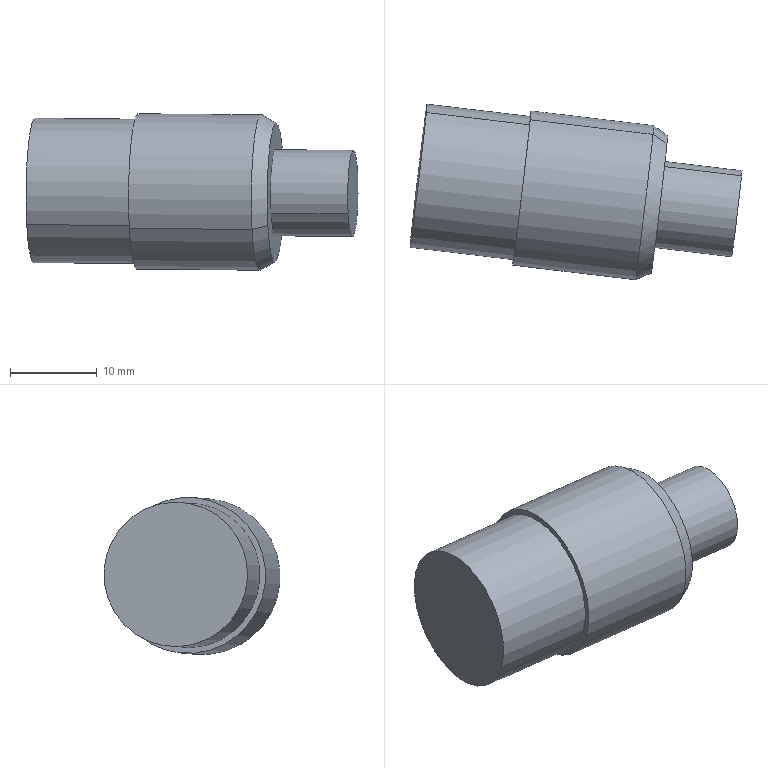Component | SolidWorks | White-1 | 1 solid | 12 faces | box 38.32 x 20.33 x 18.14 mm | volume 7353 mm3 | cylinder 6 | plane 4 | cone 2 | commonest cylinder face diameters 16.68 x2 10 x2 18 x2
build123d program:
from build123d import *

# Parameters (mm, degrees)
SKETCH1_R           = 5
BOSS_EXTRUDE1_DEPTH = 9
SKETCH2_R           = 9
BOSS_EXTRUDE2_DEPTH = 18
CHAMFER1_SIZE       = 1
CHAMFER1_SIZE2      = 1.732
CUT_EXTRUDE1_START  = -2
SKETCH3_R           = 9
SKETCH3_R_2         = 8.34
CUT_EXTRUDE1_DEPTH  = 2
SKETCH4_R           = 8.34
BOSS_EXTRUDE3_DEPTH = 10


with BuildPart() as part:
    # Sketch1 → Boss-Extrude1 (new body)
    with BuildSketch(Plane.XY):
        Circle(SKETCH1_R)
    extrude(amount=BOSS_EXTRUDE1_DEPTH)

    # Sketch2 → Boss-Extrude2 (add)
    with BuildSketch(Plane.XY.offset(9)):
        Circle(SKETCH2_R)
    extrude(amount=BOSS_EXTRUDE2_DEPTH)

    # Chamfer1
    chamfer1_edges = [part.edges().sort_by_distance(p)[0] for p in [
        (-9, 0, 9),
    ]]
    chamfer1_side = [part.faces().sort_by_distance(p)[0] for p in [
        (-8.745, 0, 9),
    ]]
    chamfer(chamfer1_edges, length=CHAMFER1_SIZE, length2=CHAMFER1_SIZE2, reference=chamfer1_side[0])

    # Sketch3 → Cut-Extrude1 (cut)
    with BuildSketch(Plane.XY.offset(27).offset(CUT_EXTRUDE1_START)):
        Circle(SKETCH3_R)
        Circle(SKETCH3_R_2, mode=Mode.SUBTRACT)
    extrude(amount=CUT_EXTRUDE1_DEPTH, mode=Mode.SUBTRACT)

    # Sketch4 → Boss-Extrude3 (add)
    with BuildSketch(Plane.XY.offset(27)):
        Circle(SKETCH4_R)
    extrude(amount=BOSS_EXTRUDE3_DEPTH)


solid = part.part

# Placed as in the assembly
solid = solid.moved(Location((-29.102, 70.681, -1.561), (-85.302, -83.182, 96.374)))
STEP:
#1=COLOUR_RGB('',0.7922,0.8196,0.9333);
#2=FILL_AREA_STYLE_COLOUR('',#1);
#3=FILL_AREA_STYLE('',(#2));
#4=SURFACE_STYLE_FILL_AREA(#3);
#5=SURFACE_SIDE_STYLE('',(#4));
#6=SURFACE_STYLE_USAGE(.BOTH.,#5);
#7=PRESENTATION_STYLE_ASSIGNMENT((#6));
#8=CARTESIAN_POINT('',(-2.087,3.186,0.1035));
#9=VERTEX_POINT('',#8);
#10=CARTESIAN_POINT('',(-2.159,2.612,-0.2072));
#11=VERTEX_POINT('',#10);
#12=CARTESIAN_POINT('',(-2.123,2.899,-0.05188));
#13=DIRECTION('',(-0.9929,0.1183,0.009724));
#14=DIRECTION('',(0.1088,0.8743,0.4731));
#15=AXIS2_PLACEMENT_3D('',#12,#13,#14);
#16=CIRCLE('',#15,0.3283);
#17=EDGE_CURVE('',#9,#11,#16,.T.);
#18=ORIENTED_EDGE('',*,*,#17,.T.);
#19=CARTESIAN_POINT('',(-2.628,2.668,-0.2026));
#20=VERTEX_POINT('',#19);
#21=CARTESIAN_POINT('',(-2.159,2.612,-0.2072));
#22=DIRECTION('',(-0.9929,0.1183,0.009724));
#23=VECTOR('',#22,39.37);
#24=LINE('',#21,#23);
#25=EDGE_CURVE('',#11,#20,#24,.T.);
#26=ORIENTED_EDGE('',*,*,#25,.T.);
#27=CARTESIAN_POINT('',(-2.556,3.242,0.108));
#28=VERTEX_POINT('',#27);
#29=CARTESIAN_POINT('',(-2.592,2.955,-0.04729));
#30=DIRECTION('',(-0.9929,0.1183,0.009724));
#31=DIRECTION('',(0.1088,0.8743,0.4731));
#32=AXIS2_PLACEMENT_3D('',#29,#30,#31);
#33=CIRCLE('',#32,0.3283);
#34=EDGE_CURVE('',#28,#20,#33,.T.);
#35=ORIENTED_EDGE('',*,*,#34,.F.);
#36=CARTESIAN_POINT('',(-2.087,3.186,0.1035));
#37=DIRECTION('',(-0.9929,0.1183,0.009724));
#38=VECTOR('',#37,39.37);
#39=LINE('',#36,#38);
#40=EDGE_CURVE('',#9,#28,#39,.T.);
#41=ORIENTED_EDGE('',*,*,#40,.F.);
#42=EDGE_LOOP('',(#18,#26,#35,#41));
#43=FACE_OUTER_BOUND('',#42,.T.);
#44=CARTESIAN_POINT('',(-2.123,2.899,-0.05188));
#45=DIRECTION('',(-0.9929,0.1183,0.009724));
#46=DIRECTION('',(0.1088,0.8743,0.4731));
#47=AXIS2_PLACEMENT_3D('',#44,#45,#46);
#48=CYLINDRICAL_SURFACE('',#47,0.3283);
#49=ADVANCED_FACE('',(#43),#48,.T.);
#50=CARTESIAN_POINT('',(-1.532,2.549,-0.207));
#51=VERTEX_POINT('',#50);
#52=CARTESIAN_POINT('',(-1.463,3.1,0.091));
#53=VERTEX_POINT('',#52);
#54=CARTESIAN_POINT('',(-1.498,2.825,-0.05801));
#55=DIRECTION('',(0.9929,-0.1183,-0.009724));
#56=DIRECTION('',(0.1088,0.8743,0.4731));
#57=AXIS2_PLACEMENT_3D('',#54,#55,#56);
#58=CIRCLE('',#57,0.315);
#59=EDGE_CURVE('',#51,#53,#58,.T.);
#60=ORIENTED_EDGE('',*,*,#59,.F.);
#61=CARTESIAN_POINT('',(-1.604,2.523,-0.225));
#62=VERTEX_POINT('',#61);
#63=CARTESIAN_POINT('',(-1.604,2.523,-0.225));
#64=DIRECTION('',(-0.9143,-0.3347,-0.2281));
#65=VECTOR('',#64,39.37);
#66=LINE('',#63,#65);
#67=EDGE_CURVE('',#51,#62,#66,.T.);
#68=ORIENTED_EDGE('',*,*,#67,.T.);
#69=CARTESIAN_POINT('',(-1.527,3.143,0.1103));
#70=VERTEX_POINT('',#69);
#71=CARTESIAN_POINT('',(-1.565,2.833,-0.05735));
#72=DIRECTION('',(-0.9929,0.1183,0.009724));
#73=DIRECTION('',(0.1088,0.8743,0.4731));
#74=AXIS2_PLACEMENT_3D('',#71,#72,#73);
#75=CIRCLE('',#74,0.3543);
#76=EDGE_CURVE('',#70,#62,#75,.T.);
#77=ORIENTED_EDGE('',*,*,#76,.F.);
#78=CARTESIAN_POINT('',(-1.527,3.143,0.1103));
#79=DIRECTION('',(-0.8055,0.5396,0.245));
#80=VECTOR('',#79,39.37);
#81=LINE('',#78,#80);
#82=EDGE_CURVE('',#53,#70,#81,.T.);
#83=ORIENTED_EDGE('',*,*,#82,.F.);
#84=EDGE_LOOP('',(#60,#68,#77,#83));
#85=FACE_OUTER_BOUND('',#84,.T.);
#86=CARTESIAN_POINT('',(-1.565,2.833,-0.05735));
#87=DIRECTION('',(-0.9929,0.1183,0.009724));
#88=DIRECTION('',(0.1088,0.8743,0.4731));
#89=AXIS2_PLACEMENT_3D('',#86,#87,#88);
#90=CONICAL_SURFACE('',#89,0.3543,0.5236);
#91=ADVANCED_FACE('',(#85),#90,.T.);
#92=CARTESIAN_POINT('',(-1.476,2.997,0.03512));
#93=VERTEX_POINT('',#92);
#94=CARTESIAN_POINT('',(-1.519,2.653,-0.1511));
#95=VERTEX_POINT('',#94);
#96=CARTESIAN_POINT('',(-1.498,2.825,-0.05801));
#97=DIRECTION('',(-0.9929,0.1183,0.009724));
#98=DIRECTION('',(0.1088,0.8743,0.4731));
#99=AXIS2_PLACEMENT_3D('',#96,#97,#98);
#100=CIRCLE('',#99,0.1969);
#101=EDGE_CURVE('',#93,#95,#100,.T.);
#102=ORIENTED_EDGE('',*,*,#101,.F.);
#103=CARTESIAN_POINT('',(-1.124,2.955,0.03167));
#104=VERTEX_POINT('',#103);
#105=CARTESIAN_POINT('',(-1.476,2.997,0.03512));
#106=DIRECTION('',(0.9929,-0.1183,-0.009724));
#107=VECTOR('',#106,39.37);
#108=LINE('',#105,#107);
#109=EDGE_CURVE('',#93,#104,#108,.T.);
#110=ORIENTED_EDGE('',*,*,#109,.T.);
#111=CARTESIAN_POINT('',(-1.167,2.611,-0.1546));
#112=VERTEX_POINT('',#111);
#113=CARTESIAN_POINT('',(-1.146,2.783,-0.06145));
#114=DIRECTION('',(-0.9929,0.1183,0.009724));
#115=DIRECTION('',(0.1088,0.8743,0.4731));
#116=AXIS2_PLACEMENT_3D('',#113,#114,#115);
#117=CIRCLE('',#116,0.1969);
#118=EDGE_CURVE('',#104,#112,#117,.T.);
#119=ORIENTED_EDGE('',*,*,#118,.T.);
#120=CARTESIAN_POINT('',(-1.519,2.653,-0.1511));
#121=DIRECTION('',(0.9929,-0.1183,-0.009724));
#122=VECTOR('',#121,39.37);
#123=LINE('',#120,#122);
#124=EDGE_CURVE('',#95,#112,#123,.T.);
#125=ORIENTED_EDGE('',*,*,#124,.F.);
#126=EDGE_LOOP('',(#102,#110,#119,#125));
#127=FACE_OUTER_BOUND('',#126,.T.);
#128=CARTESIAN_POINT('',(-1.498,2.825,-0.05801));
#129=DIRECTION('',(0.9929,-0.1183,-0.009724));
#130=DIRECTION('',(-0.1088,-0.8743,-0.4731));
#131=AXIS2_PLACEMENT_3D('',#128,#129,#130);
#132=CYLINDRICAL_SURFACE('',#131,0.1969);
#133=ADVANCED_FACE('',(#127),#132,.T.);
#134=CARTESIAN_POINT('',(-2.084,3.209,0.1157));
#135=VERTEX_POINT('',#134);
#136=CARTESIAN_POINT('',(-2.162,2.589,-0.2195));
#137=VERTEX_POINT('',#136);
#138=CARTESIAN_POINT('',(-2.123,2.899,-0.05188));
#139=DIRECTION('',(-0.9929,0.1183,0.009724));
#140=DIRECTION('',(0.1088,0.8743,0.4731));
#141=AXIS2_PLACEMENT_3D('',#138,#139,#140);
#142=CIRCLE('',#141,0.3543);
#143=EDGE_CURVE('',#135,#137,#142,.T.);
#144=ORIENTED_EDGE('',*,*,#143,.F.);
#145=CARTESIAN_POINT('',(-2.163,3.218,0.1165));
#146=DIRECTION('',(0.9929,-0.1183,-0.009724));
#147=VECTOR('',#146,39.37);
#148=LINE('',#145,#147);
#149=EDGE_CURVE('',#135,#70,#148,.T.);
#150=ORIENTED_EDGE('',*,*,#149,.T.);
#151=ORIENTED_EDGE('',*,*,#76,.T.);
#152=CARTESIAN_POINT('',(-2.24,2.599,-0.2187));
#153=DIRECTION('',(0.9929,-0.1183,-0.009724));
#154=VECTOR('',#153,39.37);
#155=LINE('',#152,#154);
#156=EDGE_CURVE('',#137,#62,#155,.T.);
#157=ORIENTED_EDGE('',*,*,#156,.F.);
#158=EDGE_LOOP('',(#144,#150,#151,#157));
#159=FACE_OUTER_BOUND('',#158,.T.);
#160=CARTESIAN_POINT('',(-2.201,2.909,-0.05112));
#161=DIRECTION('',(0.9929,-0.1183,-0.009724));
#162=DIRECTION('',(-0.1088,-0.8743,-0.4731));
#163=AXIS2_PLACEMENT_3D('',#160,#161,#162);
#164=CYLINDRICAL_SURFACE('',#163,0.3543);
#165=ADVANCED_FACE('',(#159),#164,.T.);
#166=ORIENTED_EDGE('',*,*,#149,.F.);
#167=CARTESIAN_POINT('',(-2.123,2.899,-0.05188));
#168=DIRECTION('',(-0.9929,0.1183,0.009724));
#169=DIRECTION('',(0.1088,0.8743,0.4731));
#170=AXIS2_PLACEMENT_3D('',#167,#168,#169);
#171=CIRCLE('',#170,0.3543);
#172=EDGE_CURVE('',#137,#135,#171,.T.);
#173=ORIENTED_EDGE('',*,*,#172,.F.);
#174=ORIENTED_EDGE('',*,*,#156,.T.);
#175=CARTESIAN_POINT('',(-1.565,2.833,-0.05735));
#176=DIRECTION('',(-0.9929,0.1183,0.009724));
#177=DIRECTION('',(0.1088,0.8743,0.4731));
#178=AXIS2_PLACEMENT_3D('',#175,#176,#177);
#179=CIRCLE('',#178,0.3543);
#180=EDGE_CURVE('',#62,#70,#179,.T.);
#181=ORIENTED_EDGE('',*,*,#180,.T.);
#182=EDGE_LOOP('',(#166,#173,#174,#181));
#183=FACE_OUTER_BOUND('',#182,.T.);
#184=CARTESIAN_POINT('',(-2.201,2.909,-0.05112));
#185=DIRECTION('',(0.9929,-0.1183,-0.009724));
#186=DIRECTION('',(-0.1088,-0.8743,-0.4731));
#187=AXIS2_PLACEMENT_3D('',#184,#185,#186);
#188=CYLINDRICAL_SURFACE('',#187,0.3543);
#189=ADVANCED_FACE('',(#183),#188,.T.);
#190=ORIENTED_EDGE('',*,*,#109,.F.);
#191=CARTESIAN_POINT('',(-1.498,2.825,-0.05801));
#192=DIRECTION('',(-0.9929,0.1183,0.009724));
#193=DIRECTION('',(0.1088,0.8743,0.4731));
#194=AXIS2_PLACEMENT_3D('',#191,#192,#193);
#195=CIRCLE('',#194,0.1969);
#196=EDGE_CURVE('',#95,#93,#195,.T.);
#197=ORIENTED_EDGE('',*,*,#196,.F.);
#198=ORIENTED_EDGE('',*,*,#124,.T.);
#199=CARTESIAN_POINT('',(-1.146,2.783,-0.06145));
#200=DIRECTION('',(-0.9929,0.1183,0.009724));
#201=DIRECTION('',(0.1088,0.8743,0.4731));
#202=AXIS2_PLACEMENT_3D('',#199,#200,#201);
#203=CIRCLE('',#202,0.1969);
#204=EDGE_CURVE('',#112,#104,#203,.T.);
#205=ORIENTED_EDGE('',*,*,#204,.T.);
#206=EDGE_LOOP('',(#190,#197,#198,#205));
#207=FACE_OUTER_BOUND('',#206,.T.);
#208=CARTESIAN_POINT('',(-1.498,2.825,-0.05801));
#209=DIRECTION('',(0.9929,-0.1183,-0.009724));
#210=DIRECTION('',(-0.1088,-0.8743,-0.4731));
#211=AXIS2_PLACEMENT_3D('',#208,#209,#210);
#212=CYLINDRICAL_SURFACE('',#211,0.1969);
#213=ADVANCED_FACE('',(#207),#212,.T.);
#214=ORIENTED_EDGE('',*,*,#204,.F.);
#215=ORIENTED_EDGE('',*,*,#118,.F.);
#216=EDGE_LOOP('',(#214,#215));
#217=FACE_OUTER_BOUND('',#216,.T.);
#218=CARTESIAN_POINT('',(-1.146,2.783,-0.06145));
#219=DIRECTION('',(-0.9929,0.1183,0.009724));
#220=DIRECTION('',(0.1088,0.8743,0.4731));
#221=AXIS2_PLACEMENT_3D('',#218,#219,#220);
#222=PLANE('',#221);
#223=ADVANCED_FACE('',(#217),#222,.F.);
#224=CARTESIAN_POINT('',(-1.498,2.825,-0.05801));
#225=DIRECTION('',(0.9929,-0.1183,-0.009724));
#226=DIRECTION('',(0.1088,0.8743,0.4731));
#227=AXIS2_PLACEMENT_3D('',#224,#225,#226);
#228=CIRCLE('',#227,0.315);
#229=EDGE_CURVE('',#53,#51,#228,.T.);
#230=ORIENTED_EDGE('',*,*,#229,.T.);
#231=ORIENTED_EDGE('',*,*,#59,.T.);
#232=EDGE_LOOP('',(#230,#231));
#233=FACE_OUTER_BOUND('',#232,.T.);
#234=ORIENTED_EDGE('',*,*,#196,.T.);
#235=ORIENTED_EDGE('',*,*,#101,.T.);
#236=EDGE_LOOP('',(#234,#235));
#237=FACE_BOUND('',#236,.T.);
#238=CARTESIAN_POINT('',(-1.498,2.825,-0.05801));
#239=DIRECTION('',(-0.9929,0.1183,0.009724));
#240=DIRECTION('',(0.1088,0.8743,0.4731));
#241=AXIS2_PLACEMENT_3D('',#238,#239,#240);
#242=PLANE('',#241);
#243=ADVANCED_FACE('',(#233,#237),#242,.F.);
#244=ORIENTED_EDGE('',*,*,#67,.F.);
#245=ORIENTED_EDGE('',*,*,#229,.F.);
#246=ORIENTED_EDGE('',*,*,#82,.T.);
#247=ORIENTED_EDGE('',*,*,#180,.F.);
#248=EDGE_LOOP('',(#244,#245,#246,#247));
#249=FACE_OUTER_BOUND('',#248,.T.);
#250=CARTESIAN_POINT('',(-1.565,2.833,-0.05735));
#251=DIRECTION('',(-0.9929,0.1183,0.009724));
#252=DIRECTION('',(0.1088,0.8743,0.4731));
#253=AXIS2_PLACEMENT_3D('',#250,#251,#252);
#254=CONICAL_SURFACE('',#253,0.3543,0.5236);
#255=ADVANCED_FACE('',(#249),#254,.T.);
#256=ORIENTED_EDGE('',*,*,#17,.F.);
#257=CARTESIAN_POINT('',(-2.123,2.899,-0.05188));
#258=DIRECTION('',(-0.9929,0.1183,0.009724));
#259=DIRECTION('',(0.1088,0.8743,0.4731));
#260=AXIS2_PLACEMENT_3D('',#257,#258,#259);
#261=CIRCLE('',#260,0.3283);
#262=EDGE_CURVE('',#11,#9,#261,.T.);
#263=ORIENTED_EDGE('',*,*,#262,.F.);
#264=EDGE_LOOP('',(#256,#263));
#265=FACE_BOUND('',#264,.T.);
#266=ORIENTED_EDGE('',*,*,#172,.T.);
#267=ORIENTED_EDGE('',*,*,#143,.T.);
#268=EDGE_LOOP('',(#266,#267));
#269=FACE_OUTER_BOUND('',#268,.T.);
#270=CARTESIAN_POINT('',(-2.123,2.899,-0.05188));
#271=DIRECTION('',(-0.9929,0.1183,0.009724));
#272=DIRECTION('',(0.1088,0.8743,0.4731));
#273=AXIS2_PLACEMENT_3D('',#270,#271,#272);
#274=PLANE('',#273);
#275=ADVANCED_FACE('',(#265,#269),#274,.T.);
#276=ORIENTED_EDGE('',*,*,#25,.F.);
#277=ORIENTED_EDGE('',*,*,#262,.T.);
#278=ORIENTED_EDGE('',*,*,#40,.T.);
#279=CARTESIAN_POINT('',(-2.592,2.955,-0.04729));
#280=DIRECTION('',(-0.9929,0.1183,0.009724));
#281=DIRECTION('',(0.1088,0.8743,0.4731));
#282=AXIS2_PLACEMENT_3D('',#279,#280,#281);
#283=CIRCLE('',#282,0.3283);
#284=EDGE_CURVE('',#20,#28,#283,.T.);
#285=ORIENTED_EDGE('',*,*,#284,.F.);
#286=EDGE_LOOP('',(#276,#277,#278,#285));
#287=FACE_OUTER_BOUND('',#286,.T.);
#288=CARTESIAN_POINT('',(-2.123,2.899,-0.05188));
#289=DIRECTION('',(-0.9929,0.1183,0.009724));
#290=DIRECTION('',(0.1088,0.8743,0.4731));
#291=AXIS2_PLACEMENT_3D('',#288,#289,#290);
#292=CYLINDRICAL_SURFACE('',#291,0.3283);
#293=ADVANCED_FACE('',(#287),#292,.T.);
#294=ORIENTED_EDGE('',*,*,#34,.T.);
#295=ORIENTED_EDGE('',*,*,#284,.T.);
#296=EDGE_LOOP('',(#294,#295));
#297=FACE_OUTER_BOUND('',#296,.T.);
#298=CARTESIAN_POINT('',(-2.592,2.955,-0.04729));
#299=DIRECTION('',(-0.9929,0.1183,0.009724));
#300=DIRECTION('',(0.1088,0.8743,0.4731));
#301=AXIS2_PLACEMENT_3D('',#298,#299,#300);
#302=PLANE('',#301);
#303=ADVANCED_FACE('',(#297),#302,.T.);
#304=CLOSED_SHELL('',(#49,#91,#133,#165,#189,#213,#223,#243,#255,#275,#293,#303));
#305=MANIFOLD_SOLID_BREP('',#304);
#306=STYLED_ITEM('',(#7),#305);
#307=(LENGTH_UNIT()NAMED_UNIT(*)SI_UNIT($,.METRE.));
#308=LENGTH_MEASURE_WITH_UNIT(LENGTH_MEASURE(0.0254),#307);
#309=DIMENSIONAL_EXPONENTS(1.,0.,0.,0.,0.,0.,0.);
#310=(CONVERSION_BASED_UNIT('',#308)LENGTH_UNIT()NAMED_UNIT(#309));
#311=UNCERTAINTY_MEASURE_WITH_UNIT(LENGTH_MEASURE(0.00001),#310,'','');
#312=(NAMED_UNIT(*)PLANE_ANGLE_UNIT()SI_UNIT($,.RADIAN.));
#313=(NAMED_UNIT(*)SI_UNIT($,.STERADIAN.)SOLID_ANGLE_UNIT());
#314=(GEOMETRIC_REPRESENTATION_CONTEXT(3)GLOBAL_UNCERTAINTY_ASSIGNED_CONTEXT((#311))GLOBAL_UNIT_ASSIGNED_CONTEXT((#310,#312,#313))REPRESENTATION_CONTEXT('',''));
#315=MECHANICAL_DESIGN_GEOMETRIC_PRESENTATION_REPRESENTATION('',(#306),#314);
#316=PRESENTATION_LAYER_ASSIGNMENT('','',(#306));
#317=CARTESIAN_POINT('',(0.,0.,0.));
#318=DIRECTION('',(0.,0.,1.));
#319=DIRECTION('',(1.,0.,0.));
#320=AXIS2_PLACEMENT_3D('',#317,#318,#319);
#321=(LENGTH_UNIT()NAMED_UNIT(*)SI_UNIT($,.METRE.));
#322=LENGTH_MEASURE_WITH_UNIT(LENGTH_MEASURE(0.0254),#321);
#323=DIMENSIONAL_EXPONENTS(1.,0.,0.,0.,0.,0.,0.);
#324=(CONVERSION_BASED_UNIT('',#322)LENGTH_UNIT()NAMED_UNIT(#323));
#325=UNCERTAINTY_MEASURE_WITH_UNIT(LENGTH_MEASURE(0.00001),#324,'','');
#326=(NAMED_UNIT(*)PLANE_ANGLE_UNIT()SI_UNIT($,.RADIAN.));
#327=(NAMED_UNIT(*)SI_UNIT($,.STERADIAN.)SOLID_ANGLE_UNIT());
#328=(GEOMETRIC_REPRESENTATION_CONTEXT(3)GLOBAL_UNCERTAINTY_ASSIGNED_CONTEXT((#325))GLOBAL_UNIT_ASSIGNED_CONTEXT((#324,#326,#327))REPRESENTATION_CONTEXT('',''));
#329=ADVANCED_BREP_SHAPE_REPRESENTATION('',(#305,#320),#328);